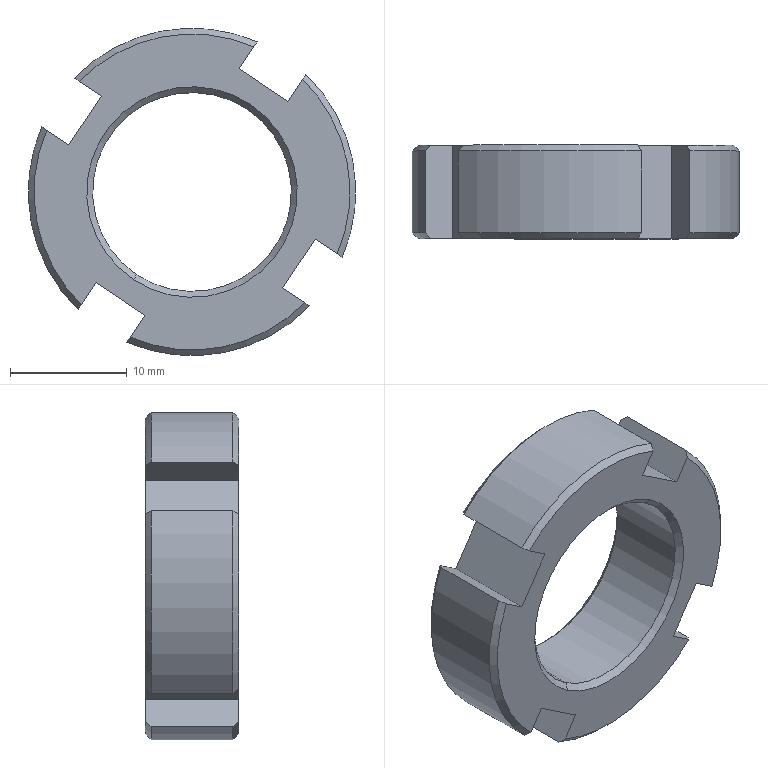Component | SolidWorks | ScrewRodFixingNut-1 | 1 solid | 32 faces | box 28 x 8 x 28 mm | volume 2612 mm3 | plane 14 | cone 12 | cylinder 6 | commonest cylinder face diameters 28 x4 17 x2
STEP:
#1=COLOUR_RGB('',0.7922,0.8196,0.9333);
#2=FILL_AREA_STYLE_COLOUR('',#1);
#3=FILL_AREA_STYLE('',(#2));
#4=SURFACE_STYLE_FILL_AREA(#3);
#5=SURFACE_SIDE_STYLE('',(#4));
#6=SURFACE_STYLE_USAGE(.BOTH.,#5);
#7=PRESENTATION_STYLE_ASSIGNMENT((#6));
#8=CARTESIAN_POINT('',(-1.348,10.043,17.753));
#9=VERTEX_POINT('',#8);
#10=CARTESIAN_POINT('',(-0.9756,10.043,18.31));
#11=VERTEX_POINT('',#10);
#12=CARTESIAN_POINT('',(-1.162,10.043,18.031));
#13=DIRECTION('',(0.,1.,0.));
#14=DIRECTION('',(0.556,0.,0.8312));
#15=AXIS2_PLACEMENT_3D('',#12,#13,#14);
#16=CIRCLE('',#15,0.3346);
#17=EDGE_CURVE('',#9,#11,#16,.T.);
#18=ORIENTED_EDGE('',*,*,#17,.F.);
#19=CARTESIAN_POINT('',(-1.359,10.063,17.737));
#20=VERTEX_POINT('',#19);
#21=CARTESIAN_POINT('',(-1.348,10.043,17.753));
#22=DIRECTION('',(-0.3931,0.7071,-0.5877));
#23=VECTOR('',#22,39.37);
#24=LINE('',#21,#23);
#25=EDGE_CURVE('',#9,#20,#24,.T.);
#26=ORIENTED_EDGE('',*,*,#25,.T.);
#27=CARTESIAN_POINT('',(-0.9647,10.063,18.326));
#28=VERTEX_POINT('',#27);
#29=CARTESIAN_POINT('',(-1.162,10.063,18.031));
#30=DIRECTION('',(0.,-1.,0.));
#31=DIRECTION('',(0.556,0.,0.8312));
#32=AXIS2_PLACEMENT_3D('',#29,#30,#31);
#33=CIRCLE('',#32,0.3543);
#34=EDGE_CURVE('',#28,#20,#33,.T.);
#35=ORIENTED_EDGE('',*,*,#34,.F.);
#36=CARTESIAN_POINT('',(-0.9756,10.043,18.31));
#37=DIRECTION('',(0.3931,0.7071,0.5877));
#38=VECTOR('',#37,39.37);
#39=LINE('',#36,#38);
#40=EDGE_CURVE('',#11,#28,#39,.T.);
#41=ORIENTED_EDGE('',*,*,#40,.F.);
#42=EDGE_LOOP('',(#18,#26,#35,#41));
#43=FACE_OUTER_BOUND('',#42,.T.);
#44=CARTESIAN_POINT('',(-1.162,10.043,18.031));
#45=DIRECTION('',(0.,1.,0.));
#46=DIRECTION('',(0.556,0.,0.8312));
#47=AXIS2_PLACEMENT_3D('',#44,#45,#46);
#48=CONICAL_SURFACE('',#47,0.3346,0.7854);
#49=ADVANCED_FACE('',(#43),#48,.F.);
#50=CARTESIAN_POINT('',(-0.9756,9.767,18.31));
#51=VERTEX_POINT('',#50);
#52=CARTESIAN_POINT('',(-1.348,9.767,17.753));
#53=VERTEX_POINT('',#52);
#54=CARTESIAN_POINT('',(-1.162,9.767,18.031));
#55=DIRECTION('',(0.,-1.,0.));
#56=DIRECTION('',(0.556,0.,0.8312));
#57=AXIS2_PLACEMENT_3D('',#54,#55,#56);
#58=CIRCLE('',#57,0.3346);
#59=EDGE_CURVE('',#51,#53,#58,.T.);
#60=ORIENTED_EDGE('',*,*,#59,.F.);
#61=CARTESIAN_POINT('',(-0.9647,9.748,18.326));
#62=VERTEX_POINT('',#61);
#63=CARTESIAN_POINT('',(-0.9647,9.748,18.326));
#64=DIRECTION('',(0.3931,-0.7071,0.5877));
#65=VECTOR('',#64,39.37);
#66=LINE('',#63,#65);
#67=EDGE_CURVE('',#51,#62,#66,.T.);
#68=ORIENTED_EDGE('',*,*,#67,.T.);
#69=CARTESIAN_POINT('',(-1.359,9.748,17.737));
#70=VERTEX_POINT('',#69);
#71=CARTESIAN_POINT('',(-1.162,9.748,18.031));
#72=DIRECTION('',(0.,1.,0.));
#73=DIRECTION('',(0.556,0.,0.8312));
#74=AXIS2_PLACEMENT_3D('',#71,#72,#73);
#75=CIRCLE('',#74,0.3543);
#76=EDGE_CURVE('',#70,#62,#75,.T.);
#77=ORIENTED_EDGE('',*,*,#76,.F.);
#78=CARTESIAN_POINT('',(-1.359,9.748,17.737));
#79=DIRECTION('',(-0.3931,-0.7071,-0.5877));
#80=VECTOR('',#79,39.37);
#81=LINE('',#78,#80);
#82=EDGE_CURVE('',#53,#70,#81,.T.);
#83=ORIENTED_EDGE('',*,*,#82,.F.);
#84=EDGE_LOOP('',(#60,#68,#77,#83));
#85=FACE_OUTER_BOUND('',#84,.T.);
#86=CARTESIAN_POINT('',(-1.162,9.748,18.031));
#87=DIRECTION('',(0.,-1.,0.));
#88=DIRECTION('',(-0.556,0.,-0.8312));
#89=AXIS2_PLACEMENT_3D('',#86,#87,#88);
#90=CONICAL_SURFACE('',#89,0.3543,0.7854);
#91=ADVANCED_FACE('',(#85),#90,.F.);
#92=ORIENTED_EDGE('',*,*,#17,.T.);
#93=CARTESIAN_POINT('',(-0.9756,10.063,18.31));
#94=DIRECTION('',(0.,-1.,0.));
#95=VECTOR('',#94,39.37);
#96=LINE('',#93,#95);
#97=EDGE_CURVE('',#11,#51,#96,.T.);
#98=ORIENTED_EDGE('',*,*,#97,.T.);
#99=ORIENTED_EDGE('',*,*,#59,.T.);
#100=CARTESIAN_POINT('',(-1.348,10.063,17.753));
#101=DIRECTION('',(0.,-1.,0.));
#102=VECTOR('',#101,39.37);
#103=LINE('',#100,#102);
#104=EDGE_CURVE('',#9,#53,#103,.T.);
#105=ORIENTED_EDGE('',*,*,#104,.F.);
#106=EDGE_LOOP('',(#92,#98,#99,#105));
#107=FACE_OUTER_BOUND('',#106,.T.);
#108=CARTESIAN_POINT('',(-1.162,10.063,18.031));
#109=DIRECTION('',(0.,-1.,0.));
#110=DIRECTION('',(-0.556,0.,-0.8312));
#111=AXIS2_PLACEMENT_3D('',#108,#109,#110);
#112=CYLINDRICAL_SURFACE('',#111,0.3346);
#113=ADVANCED_FACE('',(#107),#112,.F.);
#114=CARTESIAN_POINT('',(-0.6562,10.043,17.812));
#115=VERTEX_POINT('',#114);
#116=CARTESIAN_POINT('',(-0.7783,10.043,18.428));
#117=VERTEX_POINT('',#116);
#118=CARTESIAN_POINT('',(-1.162,10.043,18.031));
#119=DIRECTION('',(0.,-1.,0.));
#120=DIRECTION('',(0.556,0.,0.8312));
#121=AXIS2_PLACEMENT_3D('',#118,#119,#120);
#122=CIRCLE('',#121,0.5512);
#123=EDGE_CURVE('',#115,#117,#122,.T.);
#124=ORIENTED_EDGE('',*,*,#123,.T.);
#125=CARTESIAN_POINT('',(-0.7783,9.767,18.428));
#126=VERTEX_POINT('',#125);
#127=CARTESIAN_POINT('',(-0.7783,10.063,18.428));
#128=DIRECTION('',(0.,-1.,0.));
#129=VECTOR('',#128,39.37);
#130=LINE('',#127,#129);
#131=EDGE_CURVE('',#117,#126,#130,.T.);
#132=ORIENTED_EDGE('',*,*,#131,.T.);
#133=CARTESIAN_POINT('',(-0.6562,9.767,17.812));
#134=VERTEX_POINT('',#133);
#135=CARTESIAN_POINT('',(-1.162,9.767,18.031));
#136=DIRECTION('',(0.,1.,0.));
#137=DIRECTION('',(0.556,0.,0.8312));
#138=AXIS2_PLACEMENT_3D('',#135,#136,#137);
#139=CIRCLE('',#138,0.5512);
#140=EDGE_CURVE('',#126,#134,#139,.T.);
#141=ORIENTED_EDGE('',*,*,#140,.T.);
#142=CARTESIAN_POINT('',(-0.6562,10.063,17.812));
#143=DIRECTION('',(0.,1.,0.));
#144=VECTOR('',#143,39.37);
#145=LINE('',#142,#144);
#146=EDGE_CURVE('',#134,#115,#145,.T.);
#147=ORIENTED_EDGE('',*,*,#146,.T.);
#148=EDGE_LOOP('',(#124,#132,#141,#147));
#149=FACE_OUTER_BOUND('',#148,.T.);
#150=CARTESIAN_POINT('',(-1.162,10.063,18.031));
#151=DIRECTION('',(0.,-1.,0.));
#152=DIRECTION('',(-0.556,0.,-0.8312));
#153=AXIS2_PLACEMENT_3D('',#150,#151,#152);
#154=CYLINDRICAL_SURFACE('',#153,0.5512);
#155=ADVANCED_FACE('',(#149),#154,.T.);
#156=CARTESIAN_POINT('',(-1.558,9.767,18.415));
#157=VERTEX_POINT('',#156);
#158=CARTESIAN_POINT('',(-0.942,9.767,18.537));
#159=VERTEX_POINT('',#158);
#160=CARTESIAN_POINT('',(-1.162,9.767,18.031));
#161=DIRECTION('',(0.,1.,0.));
#162=DIRECTION('',(0.556,0.,0.8312));
#163=AXIS2_PLACEMENT_3D('',#160,#161,#162);
#164=CIRCLE('',#163,0.5512);
#165=EDGE_CURVE('',#157,#159,#164,.T.);
#166=ORIENTED_EDGE('',*,*,#165,.T.);
#167=CARTESIAN_POINT('',(-0.942,10.043,18.537));
#168=VERTEX_POINT('',#167);
#169=CARTESIAN_POINT('',(-0.942,10.063,18.537));
#170=DIRECTION('',(0.,1.,0.));
#171=VECTOR('',#170,39.37);
#172=LINE('',#169,#171);
#173=EDGE_CURVE('',#159,#168,#172,.T.);
#174=ORIENTED_EDGE('',*,*,#173,.T.);
#175=CARTESIAN_POINT('',(-1.558,10.043,18.415));
#176=VERTEX_POINT('',#175);
#177=CARTESIAN_POINT('',(-1.162,10.043,18.031));
#178=DIRECTION('',(0.,-1.,0.));
#179=DIRECTION('',(0.556,0.,0.8312));
#180=AXIS2_PLACEMENT_3D('',#177,#178,#179);
#181=CIRCLE('',#180,0.5512);
#182=EDGE_CURVE('',#168,#176,#181,.T.);
#183=ORIENTED_EDGE('',*,*,#182,.T.);
#184=CARTESIAN_POINT('',(-1.558,10.063,18.415));
#185=DIRECTION('',(0.,-1.,0.));
#186=VECTOR('',#185,39.37);
#187=LINE('',#184,#186);
#188=EDGE_CURVE('',#176,#157,#187,.T.);
#189=ORIENTED_EDGE('',*,*,#188,.T.);
#190=EDGE_LOOP('',(#166,#174,#183,#189));
#191=FACE_OUTER_BOUND('',#190,.T.);
#192=CARTESIAN_POINT('',(-1.162,10.063,18.031));
#193=DIRECTION('',(0.,-1.,0.));
#194=DIRECTION('',(-0.556,0.,-0.8312));
#195=AXIS2_PLACEMENT_3D('',#192,#193,#194);
#196=CYLINDRICAL_SURFACE('',#195,0.5512);
#197=ADVANCED_FACE('',(#191),#196,.T.);
#198=CARTESIAN_POINT('',(-0.7895,9.748,18.411));
#199=VERTEX_POINT('',#198);
#200=CARTESIAN_POINT('',(-0.7895,9.748,18.411));
#201=CARTESIAN_POINT('',(-0.7858,9.754,18.416));
#202=CARTESIAN_POINT('',(-0.7821,9.761,18.422));
#203=CARTESIAN_POINT('',(-0.7783,9.767,18.428));
#204=B_SPLINE_CURVE_WITH_KNOTS('',3,(#200,#201,#202,#203),.UNSPECIFIED.,.F.,.F.,(4,4),(0.005174,0.005887),.UNSPECIFIED.);
#205=EDGE_CURVE('',#199,#126,#204,.T.);
#206=ORIENTED_EDGE('',*,*,#205,.F.);
#207=CARTESIAN_POINT('',(-0.6728,9.748,17.823));
#208=VERTEX_POINT('',#207);
#209=CARTESIAN_POINT('',(-1.162,9.748,18.031));
#210=DIRECTION('',(0.,-1.,0.));
#211=DIRECTION('',(0.556,0.,0.8312));
#212=AXIS2_PLACEMENT_3D('',#209,#210,#211);
#213=CIRCLE('',#212,0.5315);
#214=EDGE_CURVE('',#208,#199,#213,.T.);
#215=ORIENTED_EDGE('',*,*,#214,.F.);
#216=CARTESIAN_POINT('',(-0.6562,9.767,17.812));
#217=CARTESIAN_POINT('',(-0.6617,9.761,17.816));
#218=CARTESIAN_POINT('',(-0.6673,9.754,17.819));
#219=CARTESIAN_POINT('',(-0.6728,9.748,17.823));
#220=B_SPLINE_CURVE_WITH_KNOTS('',3,(#216,#217,#218,#219),.UNSPECIFIED.,.F.,.F.,(4,4),(0.005322,0.006035),.UNSPECIFIED.);
#221=EDGE_CURVE('',#134,#208,#220,.T.);
#222=ORIENTED_EDGE('',*,*,#221,.F.);
#223=ORIENTED_EDGE('',*,*,#140,.F.);
#224=EDGE_LOOP('',(#206,#215,#222,#223));
#225=FACE_OUTER_BOUND('',#224,.T.);
#226=CARTESIAN_POINT('',(-1.162,9.767,18.031));
#227=DIRECTION('',(0.,1.,0.));
#228=DIRECTION('',(0.556,0.,0.8312));
#229=AXIS2_PLACEMENT_3D('',#226,#227,#228);
#230=CONICAL_SURFACE('',#229,0.5512,0.7854);
#231=ADVANCED_FACE('',(#225),#230,.T.);
#232=CARTESIAN_POINT('',(-0.9531,9.748,18.52));
#233=VERTEX_POINT('',#232);
#234=CARTESIAN_POINT('',(-0.942,9.767,18.537));
#235=CARTESIAN_POINT('',(-0.9457,9.761,18.531));
#236=CARTESIAN_POINT('',(-0.9494,9.754,18.526));
#237=CARTESIAN_POINT('',(-0.9531,9.748,18.52));
#238=B_SPLINE_CURVE_WITH_KNOTS('',3,(#234,#235,#236,#237),.UNSPECIFIED.,.F.,.F.,(4,4),(0.005322,0.006035),.UNSPECIFIED.);
#239=EDGE_CURVE('',#159,#233,#238,.T.);
#240=ORIENTED_EDGE('',*,*,#239,.F.);
#241=ORIENTED_EDGE('',*,*,#165,.F.);
#242=CARTESIAN_POINT('',(-1.541,9.748,18.404));
#243=VERTEX_POINT('',#242);
#244=CARTESIAN_POINT('',(-1.541,9.748,18.404));
#245=CARTESIAN_POINT('',(-1.547,9.754,18.407));
#246=CARTESIAN_POINT('',(-1.552,9.761,18.411));
#247=CARTESIAN_POINT('',(-1.558,9.767,18.415));
#248=B_SPLINE_CURVE_WITH_KNOTS('',3,(#244,#245,#246,#247),.UNSPECIFIED.,.F.,.F.,(4,4),(0.005174,0.005887),.UNSPECIFIED.);
#249=EDGE_CURVE('',#243,#157,#248,.T.);
#250=ORIENTED_EDGE('',*,*,#249,.F.);
#251=CARTESIAN_POINT('',(-1.162,9.748,18.031));
#252=DIRECTION('',(0.,-1.,0.));
#253=DIRECTION('',(0.556,0.,0.8312));
#254=AXIS2_PLACEMENT_3D('',#251,#252,#253);
#255=CIRCLE('',#254,0.5315);
#256=EDGE_CURVE('',#233,#243,#255,.T.);
#257=ORIENTED_EDGE('',*,*,#256,.F.);
#258=EDGE_LOOP('',(#240,#241,#250,#257));
#259=FACE_OUTER_BOUND('',#258,.T.);
#260=CARTESIAN_POINT('',(-1.162,9.767,18.031));
#261=DIRECTION('',(0.,1.,0.));
#262=DIRECTION('',(0.556,0.,0.8312));
#263=AXIS2_PLACEMENT_3D('',#260,#261,#262);
#264=CONICAL_SURFACE('',#263,0.5512,0.7854);
#265=ADVANCED_FACE('',(#259),#264,.T.);
#266=CARTESIAN_POINT('',(-0.7895,10.063,18.411));
#267=VERTEX_POINT('',#266);
#268=CARTESIAN_POINT('',(-0.7783,10.043,18.428));
#269=CARTESIAN_POINT('',(-0.7821,10.049,18.422));
#270=CARTESIAN_POINT('',(-0.7858,10.056,18.416));
#271=CARTESIAN_POINT('',(-0.7895,10.063,18.411));
#272=B_SPLINE_CURVE_WITH_KNOTS('',3,(#268,#269,#270,#271),.UNSPECIFIED.,.F.,.F.,(4,4),(0.005322,0.006035),.UNSPECIFIED.);
#273=EDGE_CURVE('',#117,#267,#272,.T.);
#274=ORIENTED_EDGE('',*,*,#273,.F.);
#275=ORIENTED_EDGE('',*,*,#123,.F.);
#276=CARTESIAN_POINT('',(-0.6728,10.063,17.823));
#277=VERTEX_POINT('',#276);
#278=CARTESIAN_POINT('',(-0.6728,10.063,17.823));
#279=CARTESIAN_POINT('',(-0.6673,10.056,17.819));
#280=CARTESIAN_POINT('',(-0.6617,10.049,17.816));
#281=CARTESIAN_POINT('',(-0.6562,10.043,17.812));
#282=B_SPLINE_CURVE_WITH_KNOTS('',3,(#278,#279,#280,#281),.UNSPECIFIED.,.F.,.F.,(4,4),(0.005174,0.005887),.UNSPECIFIED.);
#283=EDGE_CURVE('',#277,#115,#282,.T.);
#284=ORIENTED_EDGE('',*,*,#283,.F.);
#285=CARTESIAN_POINT('',(-1.162,10.063,18.031));
#286=DIRECTION('',(0.,1.,0.));
#287=DIRECTION('',(0.556,0.,0.8312));
#288=AXIS2_PLACEMENT_3D('',#285,#286,#287);
#289=CIRCLE('',#288,0.5315);
#290=EDGE_CURVE('',#267,#277,#289,.T.);
#291=ORIENTED_EDGE('',*,*,#290,.F.);
#292=EDGE_LOOP('',(#274,#275,#284,#291));
#293=FACE_OUTER_BOUND('',#292,.T.);
#294=CARTESIAN_POINT('',(-1.162,10.063,18.031));
#295=DIRECTION('',(0.,-1.,0.));
#296=DIRECTION('',(-0.556,0.,-0.8312));
#297=AXIS2_PLACEMENT_3D('',#294,#295,#296);
#298=CONICAL_SURFACE('',#297,0.5315,0.7854);
#299=ADVANCED_FACE('',(#293),#298,.T.);
#300=CARTESIAN_POINT('',(-0.9531,10.063,18.52));
#301=VERTEX_POINT('',#300);
#302=CARTESIAN_POINT('',(-0.9531,10.063,18.52));
#303=CARTESIAN_POINT('',(-0.9494,10.056,18.526));
#304=CARTESIAN_POINT('',(-0.9457,10.049,18.531));
#305=CARTESIAN_POINT('',(-0.942,10.043,18.537));
#306=B_SPLINE_CURVE_WITH_KNOTS('',3,(#302,#303,#304,#305),.UNSPECIFIED.,.F.,.F.,(4,4),(0.005174,0.005887),.UNSPECIFIED.);
#307=EDGE_CURVE('',#301,#168,#306,.T.);
#308=ORIENTED_EDGE('',*,*,#307,.F.);
#309=CARTESIAN_POINT('',(-1.541,10.063,18.404));
#310=VERTEX_POINT('',#309);
#311=CARTESIAN_POINT('',(-1.162,10.063,18.031));
#312=DIRECTION('',(0.,1.,0.));
#313=DIRECTION('',(0.556,0.,0.8312));
#314=AXIS2_PLACEMENT_3D('',#311,#312,#313);
#315=CIRCLE('',#314,0.5315);
#316=EDGE_CURVE('',#310,#301,#315,.T.);
#317=ORIENTED_EDGE('',*,*,#316,.F.);
#318=CARTESIAN_POINT('',(-1.558,10.043,18.415));
#319=CARTESIAN_POINT('',(-1.552,10.049,18.411));
#320=CARTESIAN_POINT('',(-1.547,10.056,18.407));
#321=CARTESIAN_POINT('',(-1.541,10.063,18.404));
#322=B_SPLINE_CURVE_WITH_KNOTS('',3,(#318,#319,#320,#321),.UNSPECIFIED.,.F.,.F.,(4,4),(0.005322,0.006035),.UNSPECIFIED.);
#323=EDGE_CURVE('',#176,#310,#322,.T.);
#324=ORIENTED_EDGE('',*,*,#323,.F.);
#325=ORIENTED_EDGE('',*,*,#182,.F.);
#326=EDGE_LOOP('',(#308,#317,#324,#325));
#327=FACE_OUTER_BOUND('',#326,.T.);
#328=CARTESIAN_POINT('',(-1.162,10.063,18.031));
#329=DIRECTION('',(0.,-1.,0.));
#330=DIRECTION('',(-0.556,0.,-0.8312));
#331=AXIS2_PLACEMENT_3D('',#328,#329,#330);
#332=CONICAL_SURFACE('',#331,0.5315,0.7854);
#333=ADVANCED_FACE('',(#327),#332,.T.);
#334=CARTESIAN_POINT('',(-1.381,10.043,17.526));
#335=VERTEX_POINT('',#334);
#336=CARTESIAN_POINT('',(-0.7656,10.043,17.648));
#337=VERTEX_POINT('',#336);
#338=CARTESIAN_POINT('',(-1.162,10.043,18.031));
#339=DIRECTION('',(0.,-1.,0.));
#340=DIRECTION('',(0.556,0.,0.8312));
#341=AXIS2_PLACEMENT_3D('',#338,#339,#340);
#342=CIRCLE('',#341,0.5512);
#343=EDGE_CURVE('',#335,#337,#342,.T.);
#344=ORIENTED_EDGE('',*,*,#343,.T.);
#345=CARTESIAN_POINT('',(-0.7656,9.767,17.648));
#346=VERTEX_POINT('',#345);
#347=CARTESIAN_POINT('',(-0.7656,10.063,17.648));
#348=DIRECTION('',(0.,-1.,0.));
#349=VECTOR('',#348,39.37);
#350=LINE('',#347,#349);
#351=EDGE_CURVE('',#337,#346,#350,.T.);
#352=ORIENTED_EDGE('',*,*,#351,.T.);
#353=CARTESIAN_POINT('',(-1.381,9.767,17.526));
#354=VERTEX_POINT('',#353);
#355=CARTESIAN_POINT('',(-1.162,9.767,18.031));
#356=DIRECTION('',(0.,1.,0.));
#357=DIRECTION('',(0.556,0.,0.8312));
#358=AXIS2_PLACEMENT_3D('',#355,#356,#357);
#359=CIRCLE('',#358,0.5512);
#360=EDGE_CURVE('',#346,#354,#359,.T.);
#361=ORIENTED_EDGE('',*,*,#360,.T.);
#362=CARTESIAN_POINT('',(-1.381,10.063,17.526));
#363=DIRECTION('',(0.,1.,0.));
#364=VECTOR('',#363,39.37);
#365=LINE('',#362,#364);
#366=EDGE_CURVE('',#354,#335,#365,.T.);
#367=ORIENTED_EDGE('',*,*,#366,.T.);
#368=EDGE_LOOP('',(#344,#352,#361,#367));
#369=FACE_OUTER_BOUND('',#368,.T.);
#370=CARTESIAN_POINT('',(-1.162,10.063,18.031));
#371=DIRECTION('',(0.,-1.,0.));
#372=DIRECTION('',(-0.556,0.,-0.8312));
#373=AXIS2_PLACEMENT_3D('',#370,#371,#372);
#374=CYLINDRICAL_SURFACE('',#373,0.5512);
#375=ADVANCED_FACE('',(#369),#374,.T.);
#376=CARTESIAN_POINT('',(-0.7823,9.748,17.659));
#377=VERTEX_POINT('',#376);
#378=CARTESIAN_POINT('',(-0.7823,9.748,17.659));
#379=CARTESIAN_POINT('',(-0.7767,9.754,17.656));
#380=CARTESIAN_POINT('',(-0.7712,9.761,17.652));
#381=CARTESIAN_POINT('',(-0.7656,9.767,17.648));
#382=B_SPLINE_CURVE_WITH_KNOTS('',3,(#378,#379,#380,#381),.UNSPECIFIED.,.F.,.F.,(4,4),(0.005174,0.005887),.UNSPECIFIED.);
#383=EDGE_CURVE('',#377,#346,#382,.T.);
#384=ORIENTED_EDGE('',*,*,#383,.F.);
#385=CARTESIAN_POINT('',(-1.37,9.748,17.543));
#386=VERTEX_POINT('',#385);
#387=CARTESIAN_POINT('',(-1.162,9.748,18.031));
#388=DIRECTION('',(0.,-1.,0.));
#389=DIRECTION('',(0.556,0.,0.8312));
#390=AXIS2_PLACEMENT_3D('',#387,#388,#389);
#391=CIRCLE('',#390,0.5315);
#392=EDGE_CURVE('',#386,#377,#391,.T.);
#393=ORIENTED_EDGE('',*,*,#392,.F.);
#394=CARTESIAN_POINT('',(-1.381,9.767,17.526));
#395=CARTESIAN_POINT('',(-1.378,9.761,17.532));
#396=CARTESIAN_POINT('',(-1.374,9.754,17.537));
#397=CARTESIAN_POINT('',(-1.37,9.748,17.543));
#398=B_SPLINE_CURVE_WITH_KNOTS('',3,(#394,#395,#396,#397),.UNSPECIFIED.,.F.,.F.,(4,4),(0.005322,0.006035),.UNSPECIFIED.);
#399=EDGE_CURVE('',#354,#386,#398,.T.);
#400=ORIENTED_EDGE('',*,*,#399,.F.);
#401=ORIENTED_EDGE('',*,*,#360,.F.);
#402=EDGE_LOOP('',(#384,#393,#400,#401));
#403=FACE_OUTER_BOUND('',#402,.T.);
#404=CARTESIAN_POINT('',(-1.162,9.767,18.031));
#405=DIRECTION('',(0.,1.,0.));
#406=DIRECTION('',(0.556,0.,0.8312));
#407=AXIS2_PLACEMENT_3D('',#404,#405,#406);
#408=CONICAL_SURFACE('',#407,0.5512,0.7854);
#409=ADVANCED_FACE('',(#403),#408,.T.);
#410=CARTESIAN_POINT('',(-0.7823,10.063,17.659));
#411=VERTEX_POINT('',#410);
#412=CARTESIAN_POINT('',(-0.7656,10.043,17.648));
#413=CARTESIAN_POINT('',(-0.7712,10.049,17.652));
#414=CARTESIAN_POINT('',(-0.7767,10.056,17.656));
#415=CARTESIAN_POINT('',(-0.7823,10.063,17.659));
#416=B_SPLINE_CURVE_WITH_KNOTS('',3,(#412,#413,#414,#415),.UNSPECIFIED.,.F.,.F.,(4,4),(0.005322,0.006035),.UNSPECIFIED.);
#417=EDGE_CURVE('',#337,#411,#416,.T.);
#418=ORIENTED_EDGE('',*,*,#417,.F.);
#419=ORIENTED_EDGE('',*,*,#343,.F.);
#420=CARTESIAN_POINT('',(-1.37,10.063,17.543));
#421=VERTEX_POINT('',#420);
#422=CARTESIAN_POINT('',(-1.37,10.063,17.543));
#423=CARTESIAN_POINT('',(-1.374,10.056,17.537));
#424=CARTESIAN_POINT('',(-1.378,10.049,17.532));
#425=CARTESIAN_POINT('',(-1.381,10.043,17.526));
#426=B_SPLINE_CURVE_WITH_KNOTS('',3,(#422,#423,#424,#425),.UNSPECIFIED.,.F.,.F.,(4,4),(0.005174,0.005887),.UNSPECIFIED.);
#427=EDGE_CURVE('',#421,#335,#426,.T.);
#428=ORIENTED_EDGE('',*,*,#427,.F.);
#429=CARTESIAN_POINT('',(-1.162,10.063,18.031));
#430=DIRECTION('',(0.,1.,0.));
#431=DIRECTION('',(0.556,0.,0.8312));
#432=AXIS2_PLACEMENT_3D('',#429,#430,#431);
#433=CIRCLE('',#432,0.5315);
#434=EDGE_CURVE('',#411,#421,#433,.T.);
#435=ORIENTED_EDGE('',*,*,#434,.F.);
#436=EDGE_LOOP('',(#418,#419,#428,#435));
#437=FACE_OUTER_BOUND('',#436,.T.);
#438=CARTESIAN_POINT('',(-1.162,10.063,18.031));
#439=DIRECTION('',(0.,-1.,0.));
#440=DIRECTION('',(-0.556,0.,-0.8312));
#441=AXIS2_PLACEMENT_3D('',#438,#439,#440);
#442=CONICAL_SURFACE('',#441,0.5315,0.7854);
#443=ADVANCED_FACE('',(#437),#442,.T.);
#444=ORIENTED_EDGE('',*,*,#34,.T.);
#445=CARTESIAN_POINT('',(-1.162,10.063,18.031));
#446=DIRECTION('',(0.,-1.,0.));
#447=DIRECTION('',(0.556,0.,0.8312));
#448=AXIS2_PLACEMENT_3D('',#445,#446,#447);
#449=CIRCLE('',#448,0.3543);
#450=EDGE_CURVE('',#20,#28,#449,.T.);
#451=ORIENTED_EDGE('',*,*,#450,.T.);
#452=EDGE_LOOP('',(#444,#451));
#453=FACE_BOUND('',#452,.T.);
#454=CARTESIAN_POINT('',(-0.8391,10.063,18.337));
#455=VERTEX_POINT('',#454);
#456=CARTESIAN_POINT('',(-0.6243,10.063,18.658));
#457=DIRECTION('',(-0.556,0.,-0.8312));
#458=VECTOR('',#457,39.37);
#459=LINE('',#456,#458);
#460=EDGE_CURVE('',#267,#455,#459,.T.);
#461=ORIENTED_EDGE('',*,*,#460,.F.);
#462=ORIENTED_EDGE('',*,*,#290,.T.);
#463=CARTESIAN_POINT('',(-0.747,10.063,17.873));
#464=VERTEX_POINT('',#463);
#465=CARTESIAN_POINT('',(-0.4259,10.063,17.658));
#466=DIRECTION('',(0.8312,0.,-0.556));
#467=VECTOR('',#466,39.37);
#468=LINE('',#465,#467);
#469=EDGE_CURVE('',#464,#277,#468,.T.);
#470=ORIENTED_EDGE('',*,*,#469,.F.);
#471=CARTESIAN_POINT('',(-0.8564,10.063,17.709));
#472=VERTEX_POINT('',#471);
#473=CARTESIAN_POINT('',(-0.8564,10.063,17.709));
#474=DIRECTION('',(0.556,0.,0.8312));
#475=VECTOR('',#474,39.37);
#476=LINE('',#473,#475);
#477=EDGE_CURVE('',#472,#464,#476,.T.);
#478=ORIENTED_EDGE('',*,*,#477,.F.);
#479=CARTESIAN_POINT('',(-0.5353,10.063,17.494));
#480=DIRECTION('',(-0.8312,0.,0.556));
#481=VECTOR('',#480,39.37);
#482=LINE('',#479,#481);
#483=EDGE_CURVE('',#411,#472,#482,.T.);
#484=ORIENTED_EDGE('',*,*,#483,.F.);
#485=ORIENTED_EDGE('',*,*,#434,.T.);
#486=CARTESIAN_POINT('',(-1.321,10.063,17.617));
#487=VERTEX_POINT('',#486);
#488=CARTESIAN_POINT('',(-1.535,10.063,17.296));
#489=DIRECTION('',(-0.556,0.,-0.8312));
#490=VECTOR('',#489,39.37);
#491=LINE('',#488,#490);
#492=EDGE_CURVE('',#487,#421,#491,.T.);
#493=ORIENTED_EDGE('',*,*,#492,.F.);
#494=CARTESIAN_POINT('',(-1.484,10.063,17.726));
#495=VERTEX_POINT('',#494);
#496=CARTESIAN_POINT('',(-1.484,10.063,17.726));
#497=DIRECTION('',(0.8312,0.,-0.556));
#498=VECTOR('',#497,39.37);
#499=LINE('',#496,#498);
#500=EDGE_CURVE('',#495,#487,#499,.T.);
#501=ORIENTED_EDGE('',*,*,#500,.F.);
#502=CARTESIAN_POINT('',(-1.534,10.063,17.652));
#503=VERTEX_POINT('',#502);
#504=CARTESIAN_POINT('',(-1.699,10.063,17.405));
#505=DIRECTION('',(0.556,0.,0.8312));
#506=VECTOR('',#505,39.37);
#507=LINE('',#504,#506);
#508=EDGE_CURVE('',#503,#495,#507,.T.);
#509=ORIENTED_EDGE('',*,*,#508,.F.);
#510=CARTESIAN_POINT('',(-1.651,10.063,18.24));
#511=VERTEX_POINT('',#510);
#512=CARTESIAN_POINT('',(-1.162,10.063,18.031));
#513=DIRECTION('',(0.,1.,0.));
#514=DIRECTION('',(0.556,0.,0.8312));
#515=AXIS2_PLACEMENT_3D('',#512,#513,#514);
#516=CIRCLE('',#515,0.5315);
#517=EDGE_CURVE('',#503,#511,#516,.T.);
#518=ORIENTED_EDGE('',*,*,#517,.T.);
#519=CARTESIAN_POINT('',(-1.576,10.063,18.19));
#520=VERTEX_POINT('',#519);
#521=CARTESIAN_POINT('',(-1.897,10.063,18.405));
#522=DIRECTION('',(-0.8312,0.,0.556));
#523=VECTOR('',#522,39.37);
#524=LINE('',#521,#523);
#525=EDGE_CURVE('',#520,#511,#524,.T.);
#526=ORIENTED_EDGE('',*,*,#525,.F.);
#527=CARTESIAN_POINT('',(-1.467,10.063,18.354));
#528=VERTEX_POINT('',#527);
#529=CARTESIAN_POINT('',(-1.467,10.063,18.354));
#530=DIRECTION('',(-0.556,0.,-0.8312));
#531=VECTOR('',#530,39.37);
#532=LINE('',#529,#531);
#533=EDGE_CURVE('',#528,#520,#532,.T.);
#534=ORIENTED_EDGE('',*,*,#533,.F.);
#535=CARTESIAN_POINT('',(-1.788,10.063,18.569));
#536=DIRECTION('',(0.8312,0.,-0.556));
#537=VECTOR('',#536,39.37);
#538=LINE('',#535,#537);
#539=EDGE_CURVE('',#310,#528,#538,.T.);
#540=ORIENTED_EDGE('',*,*,#539,.F.);
#541=ORIENTED_EDGE('',*,*,#316,.T.);
#542=CARTESIAN_POINT('',(-1.003,10.063,18.446));
#543=VERTEX_POINT('',#542);
#544=CARTESIAN_POINT('',(-0.7879,10.063,18.767));
#545=DIRECTION('',(0.556,0.,0.8312));
#546=VECTOR('',#545,39.37);
#547=LINE('',#544,#546);
#548=EDGE_CURVE('',#543,#301,#547,.T.);
#549=ORIENTED_EDGE('',*,*,#548,.F.);
#550=CARTESIAN_POINT('',(-0.8391,10.063,18.337));
#551=DIRECTION('',(-0.8312,0.,0.556));
#552=VECTOR('',#551,39.37);
#553=LINE('',#550,#552);
#554=EDGE_CURVE('',#455,#543,#553,.T.);
#555=ORIENTED_EDGE('',*,*,#554,.F.);
#556=EDGE_LOOP('',(#461,#462,#470,#478,#484,#485,#493,#501,#509,#518,#526,#534,#540,#541,#549,#555));
#557=FACE_OUTER_BOUND('',#556,.T.);
#558=CARTESIAN_POINT('',(-1.162,10.063,18.031));
#559=DIRECTION('',(0.,1.,0.));
#560=DIRECTION('',(0.556,0.,0.8312));
#561=AXIS2_PLACEMENT_3D('',#558,#559,#560);
#562=PLANE('',#561);
#563=ADVANCED_FACE('',(#453,#557),#562,.T.);
#564=ORIENTED_EDGE('',*,*,#76,.T.);
#565=CARTESIAN_POINT('',(-1.162,9.748,18.031));
#566=DIRECTION('',(0.,1.,0.));
#567=DIRECTION('',(0.556,0.,0.8312));
#568=AXIS2_PLACEMENT_3D('',#565,#566,#567);
#569=CIRCLE('',#568,0.3543);
#570=EDGE_CURVE('',#62,#70,#569,.T.);
#571=ORIENTED_EDGE('',*,*,#570,.T.);
#572=EDGE_LOOP('',(#564,#571));
#573=FACE_BOUND('',#572,.T.);
#574=ORIENTED_EDGE('',*,*,#214,.T.);
#575=CARTESIAN_POINT('',(-0.8391,9.748,18.337));
#576=VERTEX_POINT('',#575);
#577=CARTESIAN_POINT('',(-0.6243,9.748,18.658));
#578=DIRECTION('',(-0.556,0.,-0.8312));
#579=VECTOR('',#578,39.37);
#580=LINE('',#577,#579);
#581=EDGE_CURVE('',#199,#576,#580,.T.);
#582=ORIENTED_EDGE('',*,*,#581,.T.);
#583=CARTESIAN_POINT('',(-1.003,9.748,18.446));
#584=VERTEX_POINT('',#583);
#585=CARTESIAN_POINT('',(-0.8391,9.748,18.337));
#586=DIRECTION('',(-0.8312,0.,0.556));
#587=VECTOR('',#586,39.37);
#588=LINE('',#585,#587);
#589=EDGE_CURVE('',#576,#584,#588,.T.);
#590=ORIENTED_EDGE('',*,*,#589,.T.);
#591=CARTESIAN_POINT('',(-0.7879,9.748,18.767));
#592=DIRECTION('',(0.556,0.,0.8312));
#593=VECTOR('',#592,39.37);
#594=LINE('',#591,#593);
#595=EDGE_CURVE('',#584,#233,#594,.T.);
#596=ORIENTED_EDGE('',*,*,#595,.T.);
#597=ORIENTED_EDGE('',*,*,#256,.T.);
#598=CARTESIAN_POINT('',(-1.467,9.748,18.354));
#599=VERTEX_POINT('',#598);
#600=CARTESIAN_POINT('',(-1.788,9.748,18.569));
#601=DIRECTION('',(0.8312,0.,-0.556));
#602=VECTOR('',#601,39.37);
#603=LINE('',#600,#602);
#604=EDGE_CURVE('',#243,#599,#603,.T.);
#605=ORIENTED_EDGE('',*,*,#604,.T.);
#606=CARTESIAN_POINT('',(-1.576,9.748,18.19));
#607=VERTEX_POINT('',#606);
#608=CARTESIAN_POINT('',(-1.467,9.748,18.354));
#609=DIRECTION('',(-0.556,0.,-0.8312));
#610=VECTOR('',#609,39.37);
#611=LINE('',#608,#610);
#612=EDGE_CURVE('',#599,#607,#611,.T.);
#613=ORIENTED_EDGE('',*,*,#612,.T.);
#614=CARTESIAN_POINT('',(-1.651,9.748,18.24));
#615=VERTEX_POINT('',#614);
#616=CARTESIAN_POINT('',(-1.897,9.748,18.405));
#617=DIRECTION('',(-0.8312,0.,0.556));
#618=VECTOR('',#617,39.37);
#619=LINE('',#616,#618);
#620=EDGE_CURVE('',#607,#615,#619,.T.);
#621=ORIENTED_EDGE('',*,*,#620,.T.);
#622=CARTESIAN_POINT('',(-1.534,9.748,17.652));
#623=VERTEX_POINT('',#622);
#624=CARTESIAN_POINT('',(-1.162,9.748,18.031));
#625=DIRECTION('',(0.,-1.,0.));
#626=DIRECTION('',(0.556,0.,0.8312));
#627=AXIS2_PLACEMENT_3D('',#624,#625,#626);
#628=CIRCLE('',#627,0.5315);
#629=EDGE_CURVE('',#615,#623,#628,.T.);
#630=ORIENTED_EDGE('',*,*,#629,.T.);
#631=CARTESIAN_POINT('',(-1.484,9.748,17.726));
#632=VERTEX_POINT('',#631);
#633=CARTESIAN_POINT('',(-1.699,9.748,17.405));
#634=DIRECTION('',(0.556,0.,0.8312));
#635=VECTOR('',#634,39.37);
#636=LINE('',#633,#635);
#637=EDGE_CURVE('',#623,#632,#636,.T.);
#638=ORIENTED_EDGE('',*,*,#637,.T.);
#639=CARTESIAN_POINT('',(-1.321,9.748,17.617));
#640=VERTEX_POINT('',#639);
#641=CARTESIAN_POINT('',(-1.484,9.748,17.726));
#642=DIRECTION('',(0.8312,0.,-0.556));
#643=VECTOR('',#642,39.37);
#644=LINE('',#641,#643);
#645=EDGE_CURVE('',#632,#640,#644,.T.);
#646=ORIENTED_EDGE('',*,*,#645,.T.);
#647=CARTESIAN_POINT('',(-1.535,9.748,17.296));
#648=DIRECTION('',(-0.556,0.,-0.8312));
#649=VECTOR('',#648,39.37);
#650=LINE('',#647,#649);
#651=EDGE_CURVE('',#640,#386,#650,.T.);
#652=ORIENTED_EDGE('',*,*,#651,.T.);
#653=ORIENTED_EDGE('',*,*,#392,.T.);
#654=CARTESIAN_POINT('',(-0.8564,9.748,17.709));
#655=VERTEX_POINT('',#654);
#656=CARTESIAN_POINT('',(-0.5353,9.748,17.494));
#657=DIRECTION('',(-0.8312,0.,0.556));
#658=VECTOR('',#657,39.37);
#659=LINE('',#656,#658);
#660=EDGE_CURVE('',#377,#655,#659,.T.);
#661=ORIENTED_EDGE('',*,*,#660,.T.);
#662=CARTESIAN_POINT('',(-0.747,9.748,17.873));
#663=VERTEX_POINT('',#662);
#664=CARTESIAN_POINT('',(-0.8564,9.748,17.709));
#665=DIRECTION('',(0.556,0.,0.8312));
#666=VECTOR('',#665,39.37);
#667=LINE('',#664,#666);
#668=EDGE_CURVE('',#655,#663,#667,.T.);
#669=ORIENTED_EDGE('',*,*,#668,.T.);
#670=CARTESIAN_POINT('',(-0.4259,9.748,17.658));
#671=DIRECTION('',(0.8312,0.,-0.556));
#672=VECTOR('',#671,39.37);
#673=LINE('',#670,#672);
#674=EDGE_CURVE('',#663,#208,#673,.T.);
#675=ORIENTED_EDGE('',*,*,#674,.T.);
#676=EDGE_LOOP('',(#574,#582,#590,#596,#597,#605,#613,#621,#630,#638,#646,#652,#653,#661,#669,#675));
#677=FACE_OUTER_BOUND('',#676,.T.);
#678=CARTESIAN_POINT('',(-1.162,9.748,18.031));
#679=DIRECTION('',(0.,1.,0.));
#680=DIRECTION('',(0.556,0.,0.8312));
#681=AXIS2_PLACEMENT_3D('',#678,#679,#680);
#682=PLANE('',#681);
#683=ADVANCED_FACE('',(#573,#677),#682,.F.);
#684=CARTESIAN_POINT('',(-1.545,9.767,17.635));
#685=VERTEX_POINT('',#684);
#686=CARTESIAN_POINT('',(-1.667,9.767,18.251));
#687=VERTEX_POINT('',#686);
#688=CARTESIAN_POINT('',(-1.162,9.767,18.031));
#689=DIRECTION('',(0.,1.,0.));
#690=DIRECTION('',(0.556,0.,0.8312));
#691=AXIS2_PLACEMENT_3D('',#688,#689,#690);
#692=CIRCLE('',#691,0.5512);
#693=EDGE_CURVE('',#685,#687,#692,.T.);
#694=ORIENTED_EDGE('',*,*,#693,.T.);
#695=CARTESIAN_POINT('',(-1.667,10.043,18.251));
#696=VERTEX_POINT('',#695);
#697=CARTESIAN_POINT('',(-1.667,10.063,18.251));
#698=DIRECTION('',(0.,1.,0.));
#699=VECTOR('',#698,39.37);
#700=LINE('',#697,#699);
#701=EDGE_CURVE('',#687,#696,#700,.T.);
#702=ORIENTED_EDGE('',*,*,#701,.T.);
#703=CARTESIAN_POINT('',(-1.545,10.043,17.635));
#704=VERTEX_POINT('',#703);
#705=CARTESIAN_POINT('',(-1.162,10.043,18.031));
#706=DIRECTION('',(0.,-1.,0.));
#707=DIRECTION('',(0.556,0.,0.8312));
#708=AXIS2_PLACEMENT_3D('',#705,#706,#707);
#709=CIRCLE('',#708,0.5512);
#710=EDGE_CURVE('',#696,#704,#709,.T.);
#711=ORIENTED_EDGE('',*,*,#710,.T.);
#712=CARTESIAN_POINT('',(-1.545,10.063,17.635));
#713=DIRECTION('',(0.,-1.,0.));
#714=VECTOR('',#713,39.37);
#715=LINE('',#712,#714);
#716=EDGE_CURVE('',#704,#685,#715,.T.);
#717=ORIENTED_EDGE('',*,*,#716,.T.);
#718=EDGE_LOOP('',(#694,#702,#711,#717));
#719=FACE_OUTER_BOUND('',#718,.T.);
#720=CARTESIAN_POINT('',(-1.162,10.063,18.031));
#721=DIRECTION('',(0.,-1.,0.));
#722=DIRECTION('',(-0.556,0.,-0.8312));
#723=AXIS2_PLACEMENT_3D('',#720,#721,#722);
#724=CYLINDRICAL_SURFACE('',#723,0.5512);
#725=ADVANCED_FACE('',(#719),#724,.T.);
#726=ORIENTED_EDGE('',*,*,#97,.F.);
#727=CARTESIAN_POINT('',(-1.162,10.043,18.031));
#728=DIRECTION('',(0.,1.,0.));
#729=DIRECTION('',(0.556,0.,0.8312));
#730=AXIS2_PLACEMENT_3D('',#727,#728,#729);
#731=CIRCLE('',#730,0.3346);
#732=EDGE_CURVE('',#11,#9,#731,.T.);
#733=ORIENTED_EDGE('',*,*,#732,.T.);
#734=ORIENTED_EDGE('',*,*,#104,.T.);
#735=CARTESIAN_POINT('',(-1.162,9.767,18.031));
#736=DIRECTION('',(0.,-1.,0.));
#737=DIRECTION('',(0.556,0.,0.8312));
#738=AXIS2_PLACEMENT_3D('',#735,#736,#737);
#739=CIRCLE('',#738,0.3346);
#740=EDGE_CURVE('',#53,#51,#739,.T.);
#741=ORIENTED_EDGE('',*,*,#740,.T.);
#742=EDGE_LOOP('',(#726,#733,#734,#741));
#743=FACE_OUTER_BOUND('',#742,.T.);
#744=CARTESIAN_POINT('',(-1.162,10.063,18.031));
#745=DIRECTION('',(0.,-1.,0.));
#746=DIRECTION('',(-0.556,0.,-0.8312));
#747=AXIS2_PLACEMENT_3D('',#744,#745,#746);
#748=CYLINDRICAL_SURFACE('',#747,0.3346);
#749=ADVANCED_FACE('',(#743),#748,.F.);
#750=CARTESIAN_POINT('',(-1.667,9.767,18.251));
#751=CARTESIAN_POINT('',(-1.662,9.761,18.247));
#752=CARTESIAN_POINT('',(-1.656,9.754,18.244));
#753=CARTESIAN_POINT('',(-1.651,9.748,18.24));
#754=B_SPLINE_CURVE_WITH_KNOTS('',3,(#750,#751,#752,#753),.UNSPECIFIED.,.F.,.F.,(4,4),(0.005322,0.006035),.UNSPECIFIED.);
#755=EDGE_CURVE('',#687,#615,#754,.T.);
#756=ORIENTED_EDGE('',*,*,#755,.F.);
#757=ORIENTED_EDGE('',*,*,#693,.F.);
#758=CARTESIAN_POINT('',(-1.534,9.748,17.652));
#759=CARTESIAN_POINT('',(-1.538,9.754,17.647));
#760=CARTESIAN_POINT('',(-1.541,9.761,17.641));
#761=CARTESIAN_POINT('',(-1.545,9.767,17.635));
#762=B_SPLINE_CURVE_WITH_KNOTS('',3,(#758,#759,#760,#761),.UNSPECIFIED.,.F.,.F.,(4,4),(0.005174,0.005887),.UNSPECIFIED.);
#763=EDGE_CURVE('',#623,#685,#762,.T.);
#764=ORIENTED_EDGE('',*,*,#763,.F.);
#765=ORIENTED_EDGE('',*,*,#629,.F.);
#766=EDGE_LOOP('',(#756,#757,#764,#765));
#767=FACE_OUTER_BOUND('',#766,.T.);
#768=CARTESIAN_POINT('',(-1.162,9.767,18.031));
#769=DIRECTION('',(0.,1.,0.));
#770=DIRECTION('',(0.556,0.,0.8312));
#771=AXIS2_PLACEMENT_3D('',#768,#769,#770);
#772=CONICAL_SURFACE('',#771,0.5512,0.7854);
#773=ADVANCED_FACE('',(#767),#772,.T.);
#774=CARTESIAN_POINT('',(-1.651,10.063,18.24));
#775=CARTESIAN_POINT('',(-1.656,10.056,18.244));
#776=CARTESIAN_POINT('',(-1.662,10.049,18.247));
#777=CARTESIAN_POINT('',(-1.667,10.043,18.251));
#778=B_SPLINE_CURVE_WITH_KNOTS('',3,(#774,#775,#776,#777),.UNSPECIFIED.,.F.,.F.,(4,4),(0.005174,0.005887),.UNSPECIFIED.);
#779=EDGE_CURVE('',#511,#696,#778,.T.);
#780=ORIENTED_EDGE('',*,*,#779,.F.);
#781=ORIENTED_EDGE('',*,*,#517,.F.);
#782=CARTESIAN_POINT('',(-1.545,10.043,17.635));
#783=CARTESIAN_POINT('',(-1.541,10.049,17.641));
#784=CARTESIAN_POINT('',(-1.538,10.056,17.647));
#785=CARTESIAN_POINT('',(-1.534,10.063,17.652));
#786=B_SPLINE_CURVE_WITH_KNOTS('',3,(#782,#783,#784,#785),.UNSPECIFIED.,.F.,.F.,(4,4),(0.005322,0.006035),.UNSPECIFIED.);
#787=EDGE_CURVE('',#704,#503,#786,.T.);
#788=ORIENTED_EDGE('',*,*,#787,.F.);
#789=ORIENTED_EDGE('',*,*,#710,.F.);
#790=EDGE_LOOP('',(#780,#781,#788,#789));
#791=FACE_OUTER_BOUND('',#790,.T.);
#792=CARTESIAN_POINT('',(-1.162,10.063,18.031));
#793=DIRECTION('',(0.,-1.,0.));
#794=DIRECTION('',(-0.556,0.,-0.8312));
#795=AXIS2_PLACEMENT_3D('',#792,#793,#794);
#796=CONICAL_SURFACE('',#795,0.5315,0.7854);
#797=ADVANCED_FACE('',(#791),#796,.T.);
#798=ORIENTED_EDGE('',*,*,#763,.T.);
#799=ORIENTED_EDGE('',*,*,#716,.F.);
#800=ORIENTED_EDGE('',*,*,#787,.T.);
#801=ORIENTED_EDGE('',*,*,#508,.T.);
#802=CARTESIAN_POINT('',(-1.484,9.748,17.726));
#803=DIRECTION('',(0.,1.,0.));
#804=VECTOR('',#803,39.37);
#805=LINE('',#802,#804);
#806=EDGE_CURVE('',#632,#495,#805,.T.);
#807=ORIENTED_EDGE('',*,*,#806,.F.);
#808=ORIENTED_EDGE('',*,*,#637,.F.);
#809=EDGE_LOOP('',(#798,#799,#800,#801,#807,#808));
#810=FACE_OUTER_BOUND('',#809,.T.);
#811=CARTESIAN_POINT('',(-1.699,9.748,17.405));
#812=DIRECTION('',(-0.8312,0.,0.556));
#813=DIRECTION('',(0.556,0.,0.8312));
#814=AXIS2_PLACEMENT_3D('',#811,#812,#813);
#815=PLANE('',#814);
#816=ADVANCED_FACE('',(#810),#815,.F.);
#817=ORIENTED_EDGE('',*,*,#399,.T.);
#818=ORIENTED_EDGE('',*,*,#651,.F.);
#819=CARTESIAN_POINT('',(-1.321,9.748,17.617));
#820=DIRECTION('',(0.,1.,0.));
#821=VECTOR('',#820,39.37);
#822=LINE('',#819,#821);
#823=EDGE_CURVE('',#640,#487,#822,.T.);
#824=ORIENTED_EDGE('',*,*,#823,.T.);
#825=ORIENTED_EDGE('',*,*,#492,.T.);
#826=ORIENTED_EDGE('',*,*,#427,.T.);
#827=ORIENTED_EDGE('',*,*,#366,.F.);
#828=EDGE_LOOP('',(#817,#818,#824,#825,#826,#827));
#829=FACE_OUTER_BOUND('',#828,.T.);
#830=CARTESIAN_POINT('',(-1.535,9.748,17.296));
#831=DIRECTION('',(0.8312,0.,-0.556));
#832=DIRECTION('',(-0.556,0.,-0.8312));
#833=AXIS2_PLACEMENT_3D('',#830,#831,#832);
#834=PLANE('',#833);
#835=ADVANCED_FACE('',(#829),#834,.F.);
#836=ORIENTED_EDGE('',*,*,#500,.T.);
#837=ORIENTED_EDGE('',*,*,#823,.F.);
#838=ORIENTED_EDGE('',*,*,#645,.F.);
#839=ORIENTED_EDGE('',*,*,#806,.T.);
#840=EDGE_LOOP('',(#836,#837,#838,#839));
#841=FACE_OUTER_BOUND('',#840,.T.);
#842=CARTESIAN_POINT('',(-1.484,9.748,17.726));
#843=DIRECTION('',(0.556,0.,0.8312));
#844=DIRECTION('',(0.8312,0.,-0.556));
#845=AXIS2_PLACEMENT_3D('',#842,#843,#844);
#846=PLANE('',#845);
#847=ADVANCED_FACE('',(#841),#846,.F.);
#848=ORIENTED_EDGE('',*,*,#383,.T.);
#849=ORIENTED_EDGE('',*,*,#351,.F.);
#850=ORIENTED_EDGE('',*,*,#417,.T.);
#851=ORIENTED_EDGE('',*,*,#483,.T.);
#852=CARTESIAN_POINT('',(-0.8564,9.748,17.709));
#853=DIRECTION('',(0.,1.,0.));
#854=VECTOR('',#853,39.37);
#855=LINE('',#852,#854);
#856=EDGE_CURVE('',#655,#472,#855,.T.);
#857=ORIENTED_EDGE('',*,*,#856,.F.);
#858=ORIENTED_EDGE('',*,*,#660,.F.);
#859=EDGE_LOOP('',(#848,#849,#850,#851,#857,#858));
#860=FACE_OUTER_BOUND('',#859,.T.);
#861=CARTESIAN_POINT('',(-0.5353,9.748,17.494));
#862=DIRECTION('',(-0.556,0.,-0.8312));
#863=DIRECTION('',(-0.8312,0.,0.556));
#864=AXIS2_PLACEMENT_3D('',#861,#862,#863);
#865=PLANE('',#864);
#866=ADVANCED_FACE('',(#860),#865,.F.);
#867=ORIENTED_EDGE('',*,*,#221,.T.);
#868=ORIENTED_EDGE('',*,*,#674,.F.);
#869=CARTESIAN_POINT('',(-0.747,9.748,17.873));
#870=DIRECTION('',(0.,1.,0.));
#871=VECTOR('',#870,39.37);
#872=LINE('',#869,#871);
#873=EDGE_CURVE('',#663,#464,#872,.T.);
#874=ORIENTED_EDGE('',*,*,#873,.T.);
#875=ORIENTED_EDGE('',*,*,#469,.T.);
#876=ORIENTED_EDGE('',*,*,#283,.T.);
#877=ORIENTED_EDGE('',*,*,#146,.F.);
#878=EDGE_LOOP('',(#867,#868,#874,#875,#876,#877));
#879=FACE_OUTER_BOUND('',#878,.T.);
#880=CARTESIAN_POINT('',(-0.4259,9.748,17.658));
#881=DIRECTION('',(0.556,0.,0.8312));
#882=DIRECTION('',(0.8312,0.,-0.556));
#883=AXIS2_PLACEMENT_3D('',#880,#881,#882);
#884=PLANE('',#883);
#885=ADVANCED_FACE('',(#879),#884,.F.);
#886=ORIENTED_EDGE('',*,*,#477,.T.);
#887=ORIENTED_EDGE('',*,*,#873,.F.);
#888=ORIENTED_EDGE('',*,*,#668,.F.);
#889=ORIENTED_EDGE('',*,*,#856,.T.);
#890=EDGE_LOOP('',(#886,#887,#888,#889));
#891=FACE_OUTER_BOUND('',#890,.T.);
#892=CARTESIAN_POINT('',(-0.8564,9.748,17.709));
#893=DIRECTION('',(-0.8312,0.,0.556));
#894=DIRECTION('',(0.556,0.,0.8312));
#895=AXIS2_PLACEMENT_3D('',#892,#893,#894);
#896=PLANE('',#895);
#897=ADVANCED_FACE('',(#891),#896,.F.);
#898=ORIENTED_EDGE('',*,*,#249,.T.);
#899=ORIENTED_EDGE('',*,*,#188,.F.);
#900=ORIENTED_EDGE('',*,*,#323,.T.);
#901=ORIENTED_EDGE('',*,*,#539,.T.);
#902=CARTESIAN_POINT('',(-1.467,9.748,18.354));
#903=DIRECTION('',(0.,1.,0.));
#904=VECTOR('',#903,39.37);
#905=LINE('',#902,#904);
#906=EDGE_CURVE('',#599,#528,#905,.T.);
#907=ORIENTED_EDGE('',*,*,#906,.F.);
#908=ORIENTED_EDGE('',*,*,#604,.F.);
#909=EDGE_LOOP('',(#898,#899,#900,#901,#907,#908));
#910=FACE_OUTER_BOUND('',#909,.T.);
#911=CARTESIAN_POINT('',(-1.788,9.748,18.569));
#912=DIRECTION('',(0.556,0.,0.8312));
#913=DIRECTION('',(0.8312,0.,-0.556));
#914=AXIS2_PLACEMENT_3D('',#911,#912,#913);
#915=PLANE('',#914);
#916=ADVANCED_FACE('',(#910),#915,.F.);
#917=ORIENTED_EDGE('',*,*,#755,.T.);
#918=ORIENTED_EDGE('',*,*,#620,.F.);
#919=CARTESIAN_POINT('',(-1.576,9.748,18.19));
#920=DIRECTION('',(0.,1.,0.));
#921=VECTOR('',#920,39.37);
#922=LINE('',#919,#921);
#923=EDGE_CURVE('',#607,#520,#922,.T.);
#924=ORIENTED_EDGE('',*,*,#923,.T.);
#925=ORIENTED_EDGE('',*,*,#525,.T.);
#926=ORIENTED_EDGE('',*,*,#779,.T.);
#927=ORIENTED_EDGE('',*,*,#701,.F.);
#928=EDGE_LOOP('',(#917,#918,#924,#925,#926,#927));
#929=FACE_OUTER_BOUND('',#928,.T.);
#930=CARTESIAN_POINT('',(-1.897,9.748,18.405));
#931=DIRECTION('',(-0.556,0.,-0.8312));
#932=DIRECTION('',(-0.8312,0.,0.556));
#933=AXIS2_PLACEMENT_3D('',#930,#931,#932);
#934=PLANE('',#933);
#935=ADVANCED_FACE('',(#929),#934,.F.);
#936=ORIENTED_EDGE('',*,*,#533,.T.);
#937=ORIENTED_EDGE('',*,*,#923,.F.);
#938=ORIENTED_EDGE('',*,*,#612,.F.);
#939=ORIENTED_EDGE('',*,*,#906,.T.);
#940=EDGE_LOOP('',(#936,#937,#938,#939));
#941=FACE_OUTER_BOUND('',#940,.T.);
#942=CARTESIAN_POINT('',(-1.467,9.748,18.354));
#943=DIRECTION('',(0.8312,0.,-0.556));
#944=DIRECTION('',(-0.556,0.,-0.8312));
#945=AXIS2_PLACEMENT_3D('',#942,#943,#944);
#946=PLANE('',#945);
#947=ADVANCED_FACE('',(#941),#946,.F.);
#948=ORIENTED_EDGE('',*,*,#205,.T.);
#949=ORIENTED_EDGE('',*,*,#131,.F.);
#950=ORIENTED_EDGE('',*,*,#273,.T.);
#951=ORIENTED_EDGE('',*,*,#460,.T.);
#952=CARTESIAN_POINT('',(-0.8391,9.748,18.337));
#953=DIRECTION('',(0.,1.,0.));
#954=VECTOR('',#953,39.37);
#955=LINE('',#952,#954);
#956=EDGE_CURVE('',#576,#455,#955,.T.);
#957=ORIENTED_EDGE('',*,*,#956,.F.);
#958=ORIENTED_EDGE('',*,*,#581,.F.);
#959=EDGE_LOOP('',(#948,#949,#950,#951,#957,#958));
#960=FACE_OUTER_BOUND('',#959,.T.);
#961=CARTESIAN_POINT('',(-0.6243,9.748,18.658));
#962=DIRECTION('',(0.8312,0.,-0.556));
#963=DIRECTION('',(-0.556,0.,-0.8312));
#964=AXIS2_PLACEMENT_3D('',#961,#962,#963);
#965=PLANE('',#964);
#966=ADVANCED_FACE('',(#960),#965,.F.);
#967=ORIENTED_EDGE('',*,*,#239,.T.);
#968=ORIENTED_EDGE('',*,*,#595,.F.);
#969=CARTESIAN_POINT('',(-1.003,9.748,18.446));
#970=DIRECTION('',(0.,1.,0.));
#971=VECTOR('',#970,39.37);
#972=LINE('',#969,#971);
#973=EDGE_CURVE('',#584,#543,#972,.T.);
#974=ORIENTED_EDGE('',*,*,#973,.T.);
#975=ORIENTED_EDGE('',*,*,#548,.T.);
#976=ORIENTED_EDGE('',*,*,#307,.T.);
#977=ORIENTED_EDGE('',*,*,#173,.F.);
#978=EDGE_LOOP('',(#967,#968,#974,#975,#976,#977));
#979=FACE_OUTER_BOUND('',#978,.T.);
#980=CARTESIAN_POINT('',(-0.7879,9.748,18.767));
#981=DIRECTION('',(-0.8312,0.,0.556));
#982=DIRECTION('',(0.556,0.,0.8312));
#983=AXIS2_PLACEMENT_3D('',#980,#981,#982);
#984=PLANE('',#983);
#985=ADVANCED_FACE('',(#979),#984,.F.);
#986=ORIENTED_EDGE('',*,*,#554,.T.);
#987=ORIENTED_EDGE('',*,*,#973,.F.);
#988=ORIENTED_EDGE('',*,*,#589,.F.);
#989=ORIENTED_EDGE('',*,*,#956,.T.);
#990=EDGE_LOOP('',(#986,#987,#988,#989));
#991=FACE_OUTER_BOUND('',#990,.T.);
#992=CARTESIAN_POINT('',(-0.8391,9.748,18.337));
#993=DIRECTION('',(-0.556,0.,-0.8312));
#994=DIRECTION('',(-0.8312,0.,0.556));
#995=AXIS2_PLACEMENT_3D('',#992,#993,#994);
#996=PLANE('',#995);
#997=ADVANCED_FACE('',(#991),#996,.F.);
#998=ORIENTED_EDGE('',*,*,#67,.F.);
#999=ORIENTED_EDGE('',*,*,#740,.F.);
#1000=ORIENTED_EDGE('',*,*,#82,.T.);
#1001=ORIENTED_EDGE('',*,*,#570,.F.);
#1002=EDGE_LOOP('',(#998,#999,#1000,#1001));
#1003=FACE_OUTER_BOUND('',#1002,.T.);
#1004=CARTESIAN_POINT('',(-1.162,9.748,18.031));
#1005=DIRECTION('',(0.,-1.,0.));
#1006=DIRECTION('',(-0.556,0.,-0.8312));
#1007=AXIS2_PLACEMENT_3D('',#1004,#1005,#1006);
#1008=CONICAL_SURFACE('',#1007,0.3543,0.7854);
#1009=ADVANCED_FACE('',(#1003),#1008,.F.);
#1010=ORIENTED_EDGE('',*,*,#25,.F.);
#1011=ORIENTED_EDGE('',*,*,#732,.F.);
#1012=ORIENTED_EDGE('',*,*,#40,.T.);
#1013=ORIENTED_EDGE('',*,*,#450,.F.);
#1014=EDGE_LOOP('',(#1010,#1011,#1012,#1013));
#1015=FACE_OUTER_BOUND('',#1014,.T.);
#1016=CARTESIAN_POINT('',(-1.162,10.043,18.031));
#1017=DIRECTION('',(0.,1.,0.));
#1018=DIRECTION('',(0.556,0.,0.8312));
#1019=AXIS2_PLACEMENT_3D('',#1016,#1017,#1018);
#1020=CONICAL_SURFACE('',#1019,0.3346,0.7854);
#1021=ADVANCED_FACE('',(#1015),#1020,.F.);
#1022=CLOSED_SHELL('',(#49,#91,#113,#155,#197,#231,#265,#299,#333,#375,#409,#443,#563,#683,#725,#749,#773,#797,#816,#835,#847,#866,#885,#897,#916,#935,#947,#966,#985,#997,#1009,#1021));
#1023=MANIFOLD_SOLID_BREP('',#1022);
#1024=STYLED_ITEM('',(#7),#1023);
#1025=(LENGTH_UNIT()NAMED_UNIT(*)SI_UNIT($,.METRE.));
#1026=LENGTH_MEASURE_WITH_UNIT(LENGTH_MEASURE(0.0254),#1025);
#1027=DIMENSIONAL_EXPONENTS(1.,0.,0.,0.,0.,0.,0.);
#1028=(CONVERSION_BASED_UNIT('',#1026)LENGTH_UNIT()NAMED_UNIT(#1027));
#1029=UNCERTAINTY_MEASURE_WITH_UNIT(LENGTH_MEASURE(0.00001),#1028,'','');
#1030=(NAMED_UNIT(*)PLANE_ANGLE_UNIT()SI_UNIT($,.RADIAN.));
#1031=(NAMED_UNIT(*)SI_UNIT($,.STERADIAN.)SOLID_ANGLE_UNIT());
#1032=(GEOMETRIC_REPRESENTATION_CONTEXT(3)GLOBAL_UNCERTAINTY_ASSIGNED_CONTEXT((#1029))GLOBAL_UNIT_ASSIGNED_CONTEXT((#1028,#1030,#1031))REPRESENTATION_CONTEXT('',''));
#1033=MECHANICAL_DESIGN_GEOMETRIC_PRESENTATION_REPRESENTATION('',(#1024),#1032);
#1034=CARTESIAN_POINT('',(0.,0.,0.));
#1035=DIRECTION('',(0.,0.,1.));
#1036=DIRECTION('',(1.,0.,0.));
#1037=AXIS2_PLACEMENT_3D('',#1034,#1035,#1036);
#1038=(LENGTH_UNIT()NAMED_UNIT(*)SI_UNIT($,.METRE.));
#1039=LENGTH_MEASURE_WITH_UNIT(LENGTH_MEASURE(0.0254),#1038);
#1040=DIMENSIONAL_EXPONENTS(1.,0.,0.,0.,0.,0.,0.);
#1041=(CONVERSION_BASED_UNIT('',#1039)LENGTH_UNIT()NAMED_UNIT(#1040));
#1042=UNCERTAINTY_MEASURE_WITH_UNIT(LENGTH_MEASURE(0.00001),#1041,'','');
#1043=(NAMED_UNIT(*)PLANE_ANGLE_UNIT()SI_UNIT($,.RADIAN.));
#1044=(NAMED_UNIT(*)SI_UNIT($,.STERADIAN.)SOLID_ANGLE_UNIT());
#1045=(GEOMETRIC_REPRESENTATION_CONTEXT(3)GLOBAL_UNCERTAINTY_ASSIGNED_CONTEXT((#1042))GLOBAL_UNIT_ASSIGNED_CONTEXT((#1041,#1043,#1044))REPRESENTATION_CONTEXT('',''));
#1046=ADVANCED_BREP_SHAPE_REPRESENTATION('',(#1023,#1037),#1045);
#1047=PRESENTATION_LAYER_ASSIGNMENT('','',(#1024));